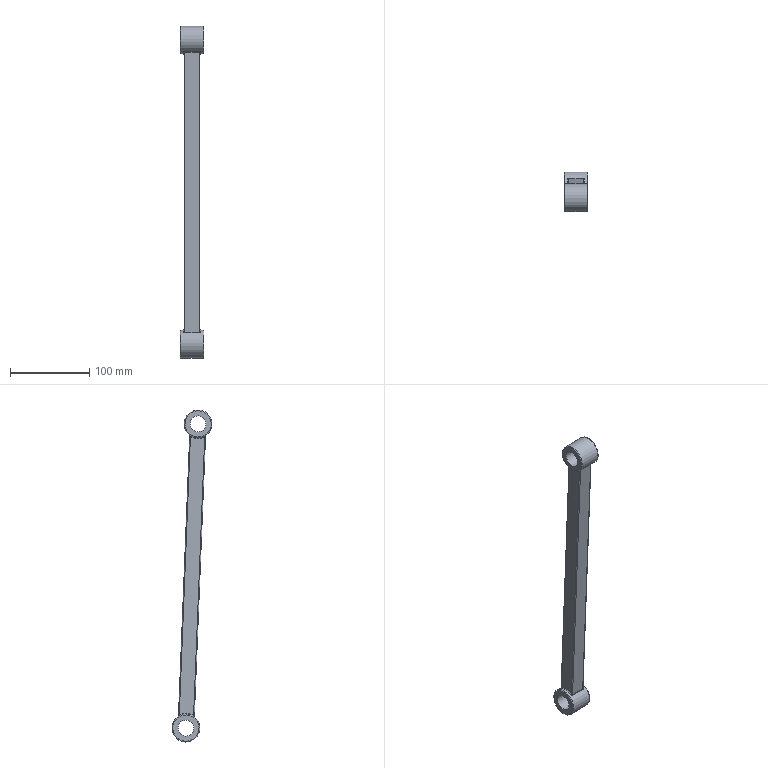Component | NX | CCJ-006 | 1 solid | 36 faces | volume 178505 mm3 | cylinder 12 | plane 8 | torus 8 | spline 8 | commonest cylinder face diameters 2 x8 35 x2 20 x2